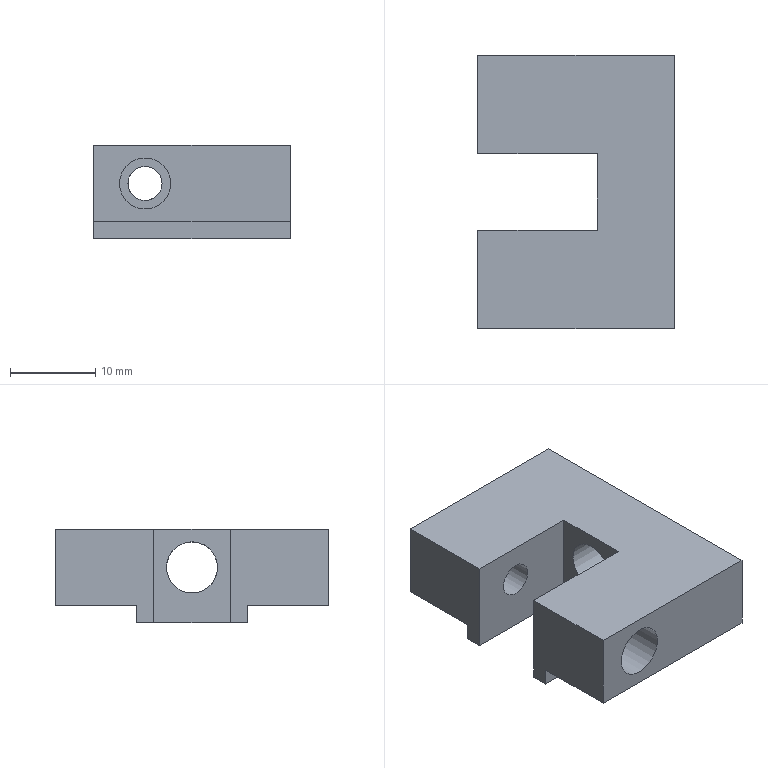Component | NX | SLIDER | 1 solid | 19 faces | volume 5167 mm3 | plane 15 | cylinder 4 | commonest cylinder face diameters 6 x2 4 x2